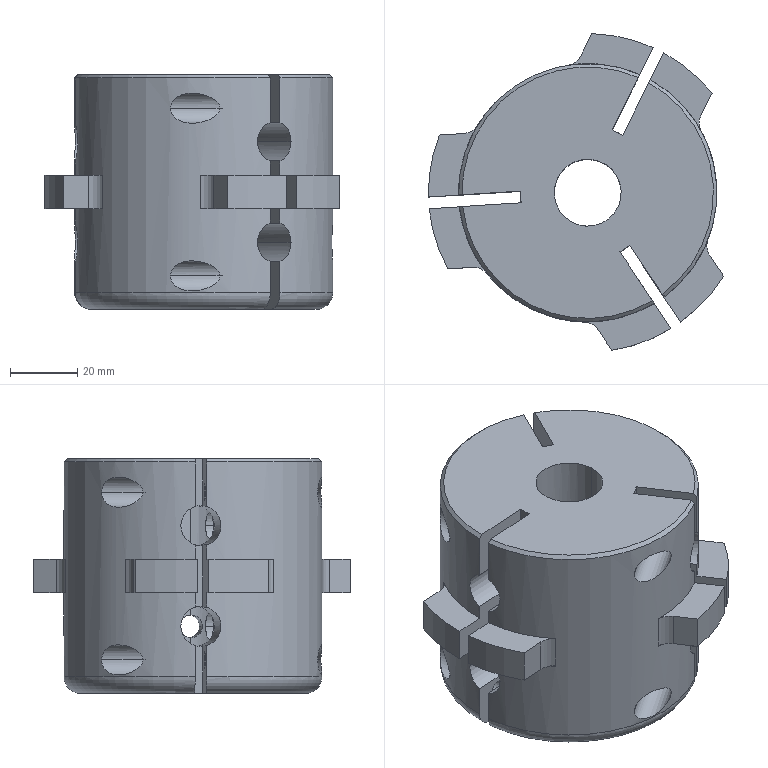Component | SolidWorks | YX-04-107GluePaperFeedingExpansionAxis-1 | 1 solid | 173 faces | volume 273310 mm3 | cylinder 71 | plane 54 | cone 45 | torus 3 | commonest cylinder face diameters 4.2 x12 9 x12 5.5 x12 12 x12 10 x8 95 x6 77 x3 14 x2 | material 45#Steel